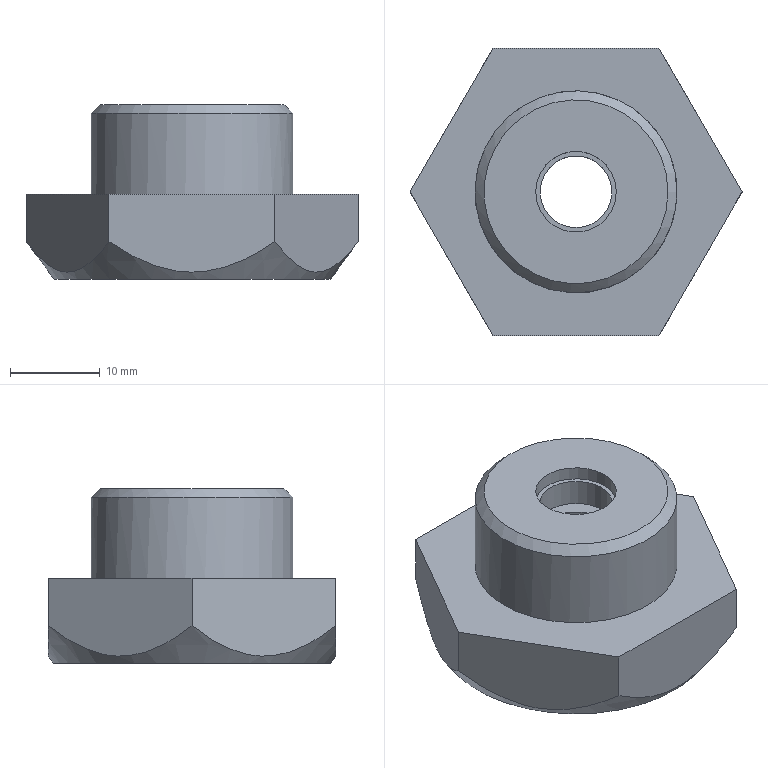Component | NX | NUT | 1 solid | 20 faces | volume 10469 mm3 | plane 12 | cylinder 5 | cone 3 | commonest cylinder face diameters 8 x1 22.5 x1 10.3 x1 16 x1 9 x1